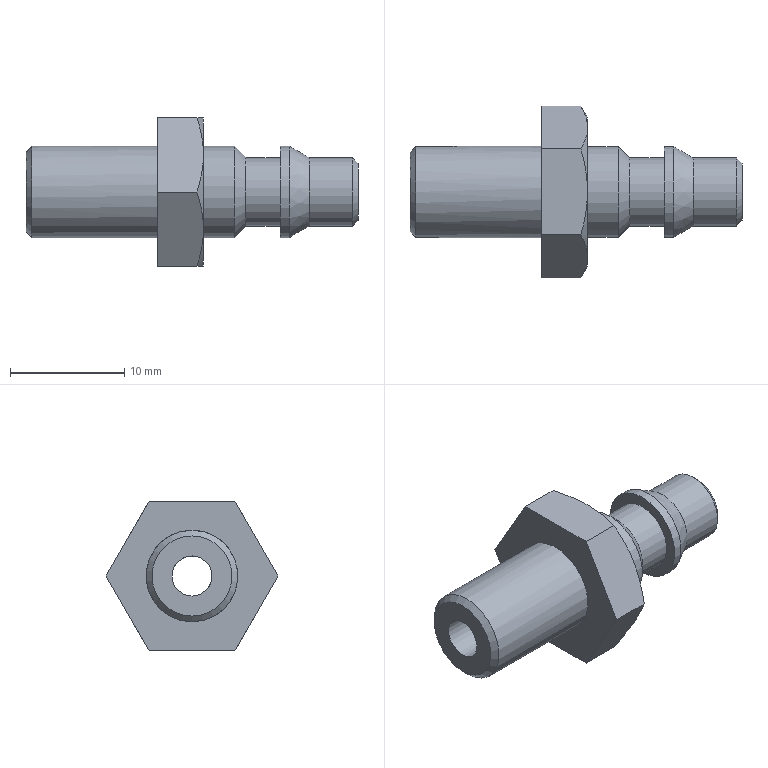Component | NX | TUBE_CONNECTOR | 1 solid | 27 faces | volume 1364 mm3 | plane 11 | cone 10 | cylinder 6 | commonest cylinder face diameters 8 x3 6 x2 3.5 x1